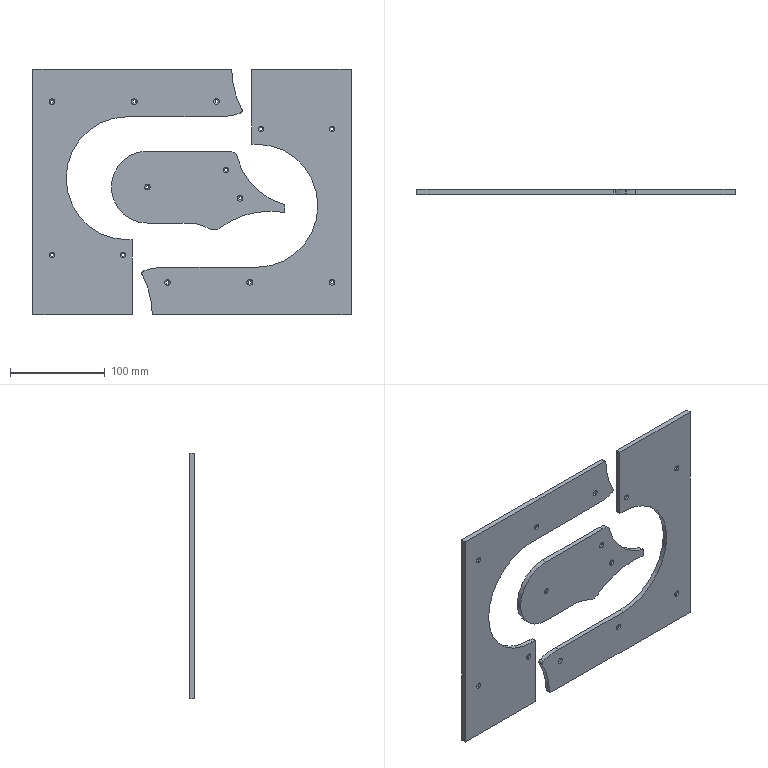CAM job | Mastercam | mm | 4 operations | part box 336 x 5 x 259
1. Contour (Ramp) | 3 - 3 平铣刀
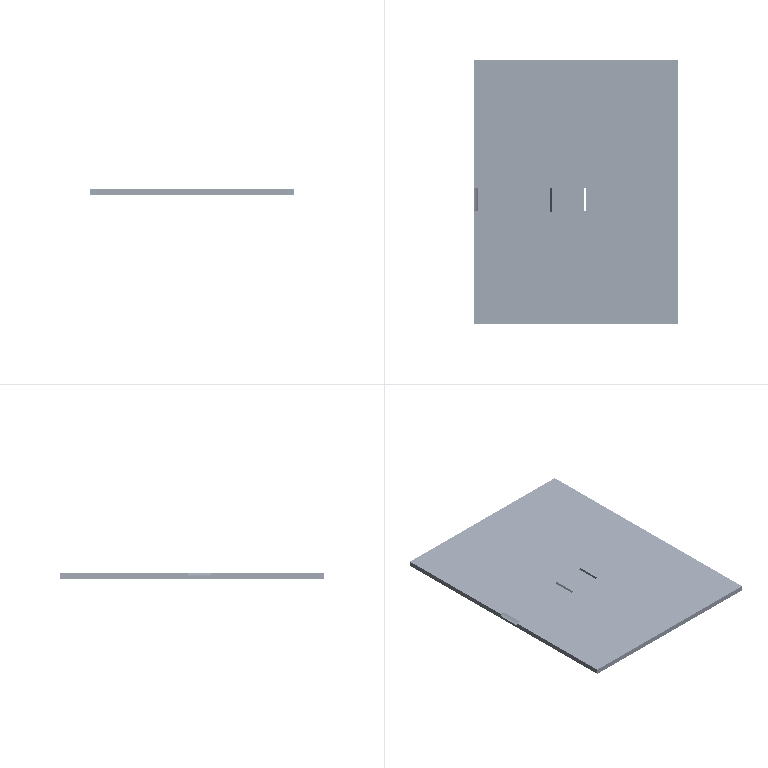2. Contour (2D) | 3 - 3 平铣刀
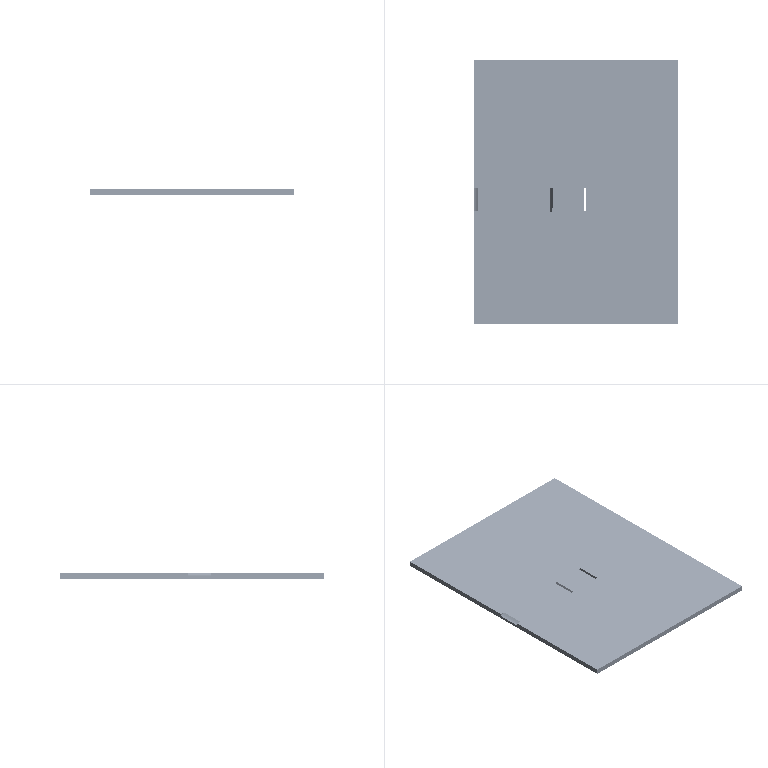3. Contour (2D chamfer) | 7 - 4 倒角刀
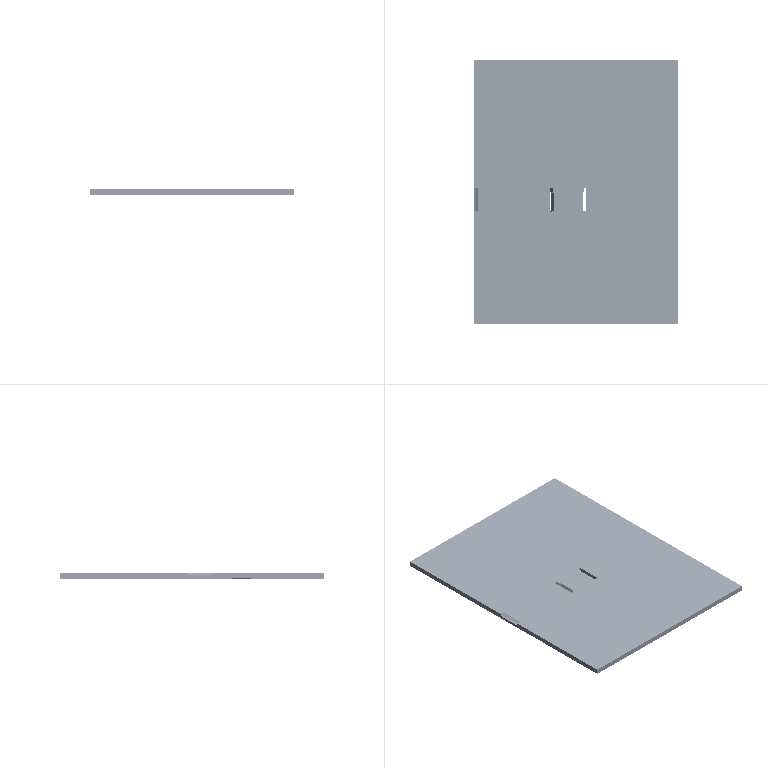4. Drill/Counterbore | 7 - 4 倒角刀